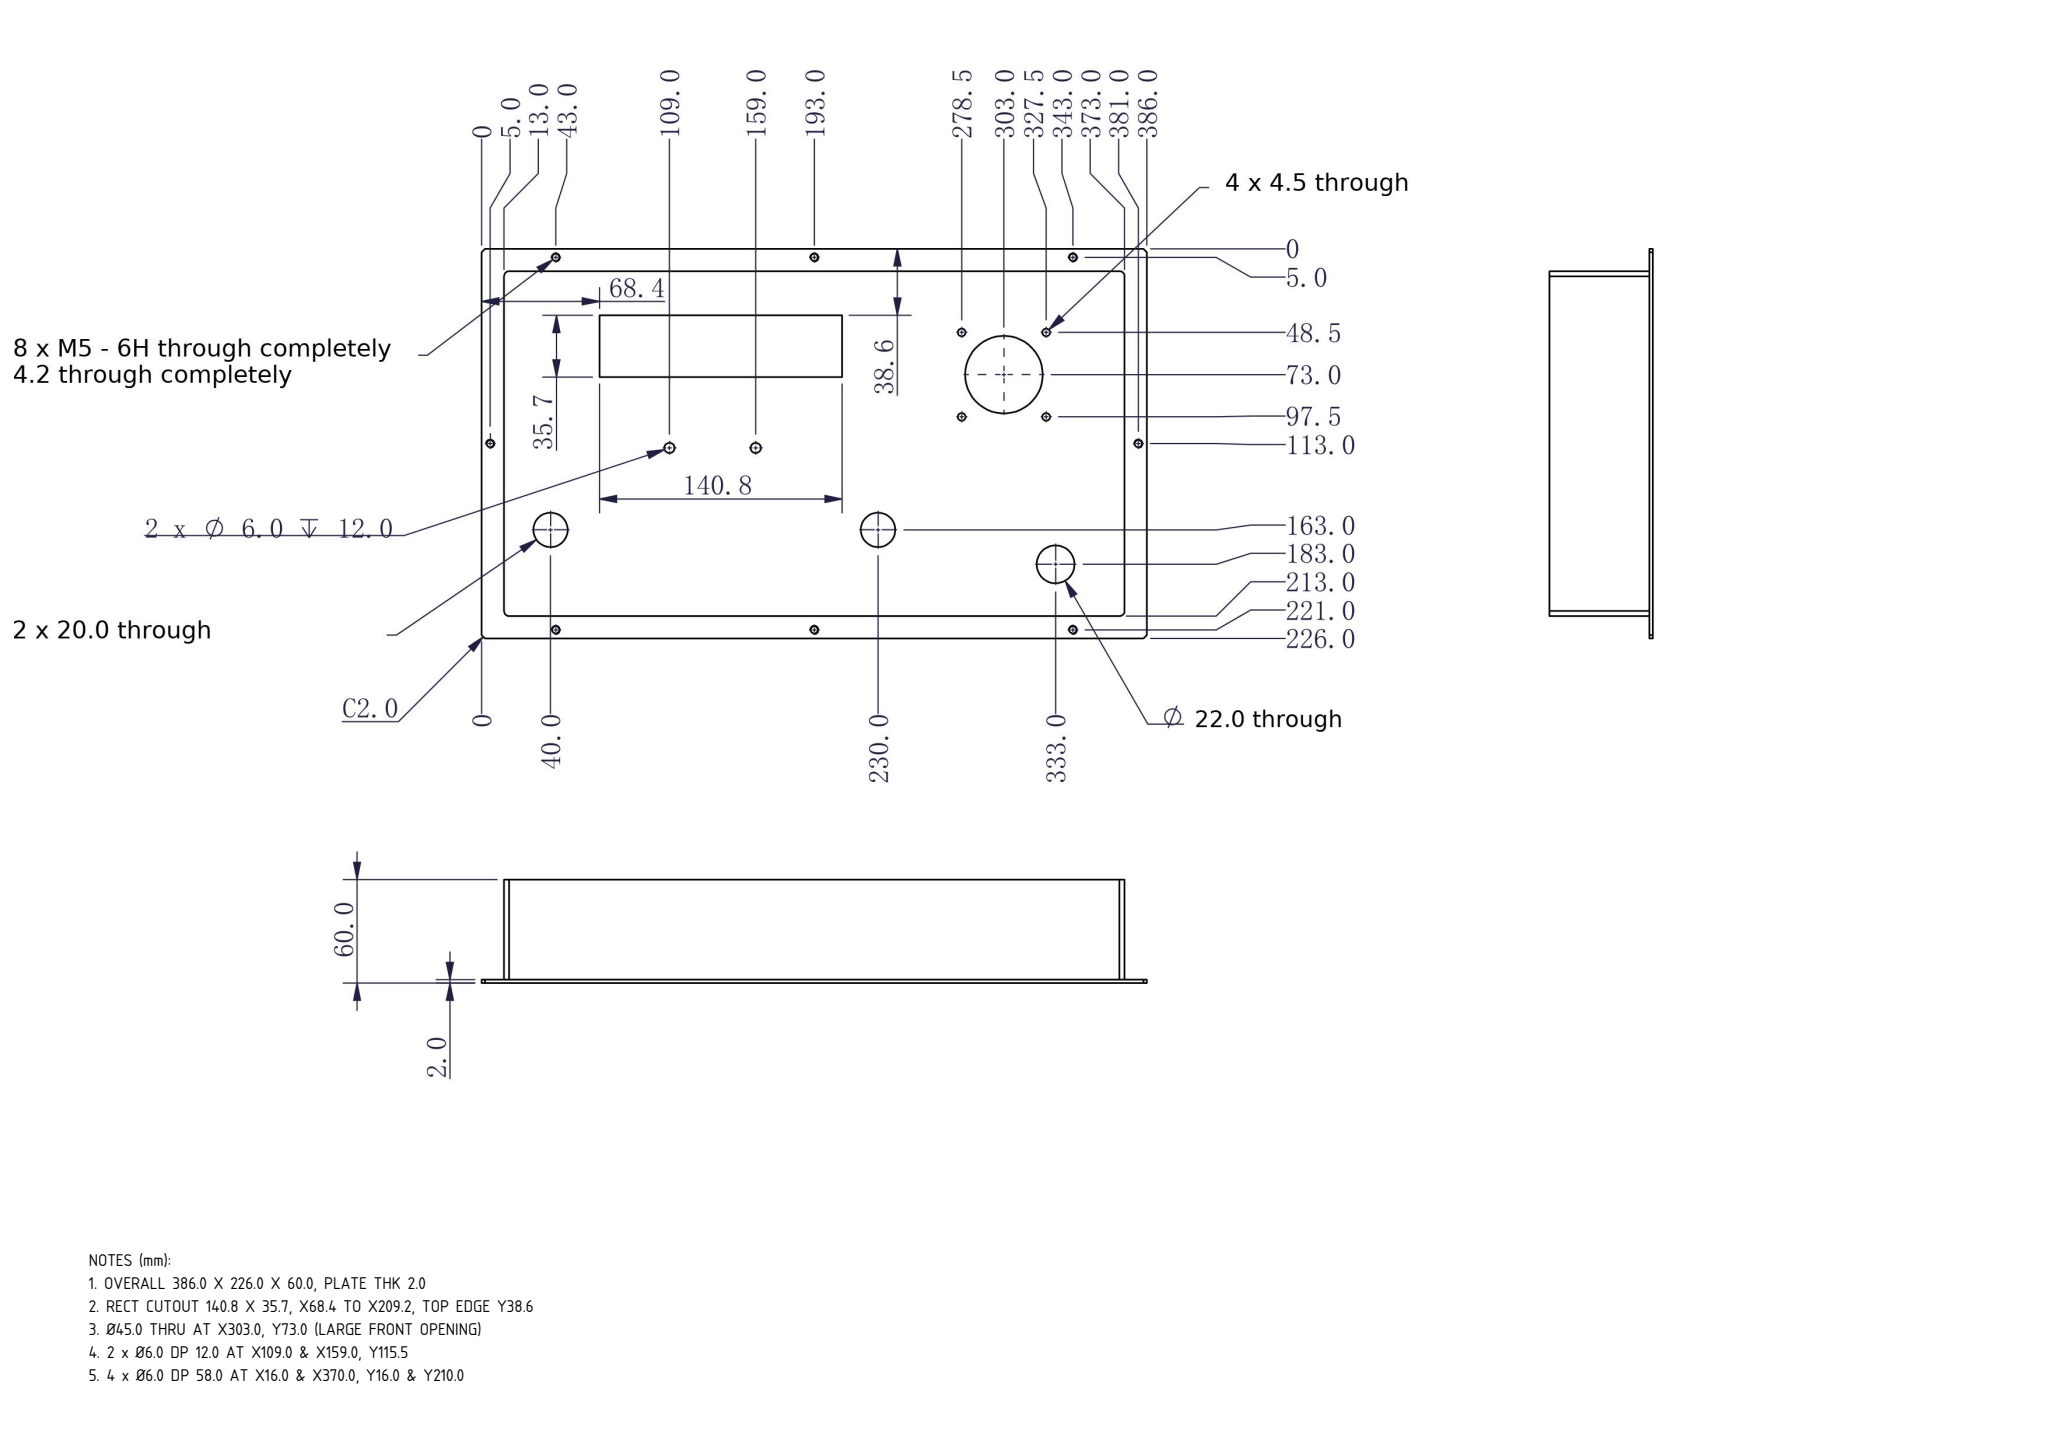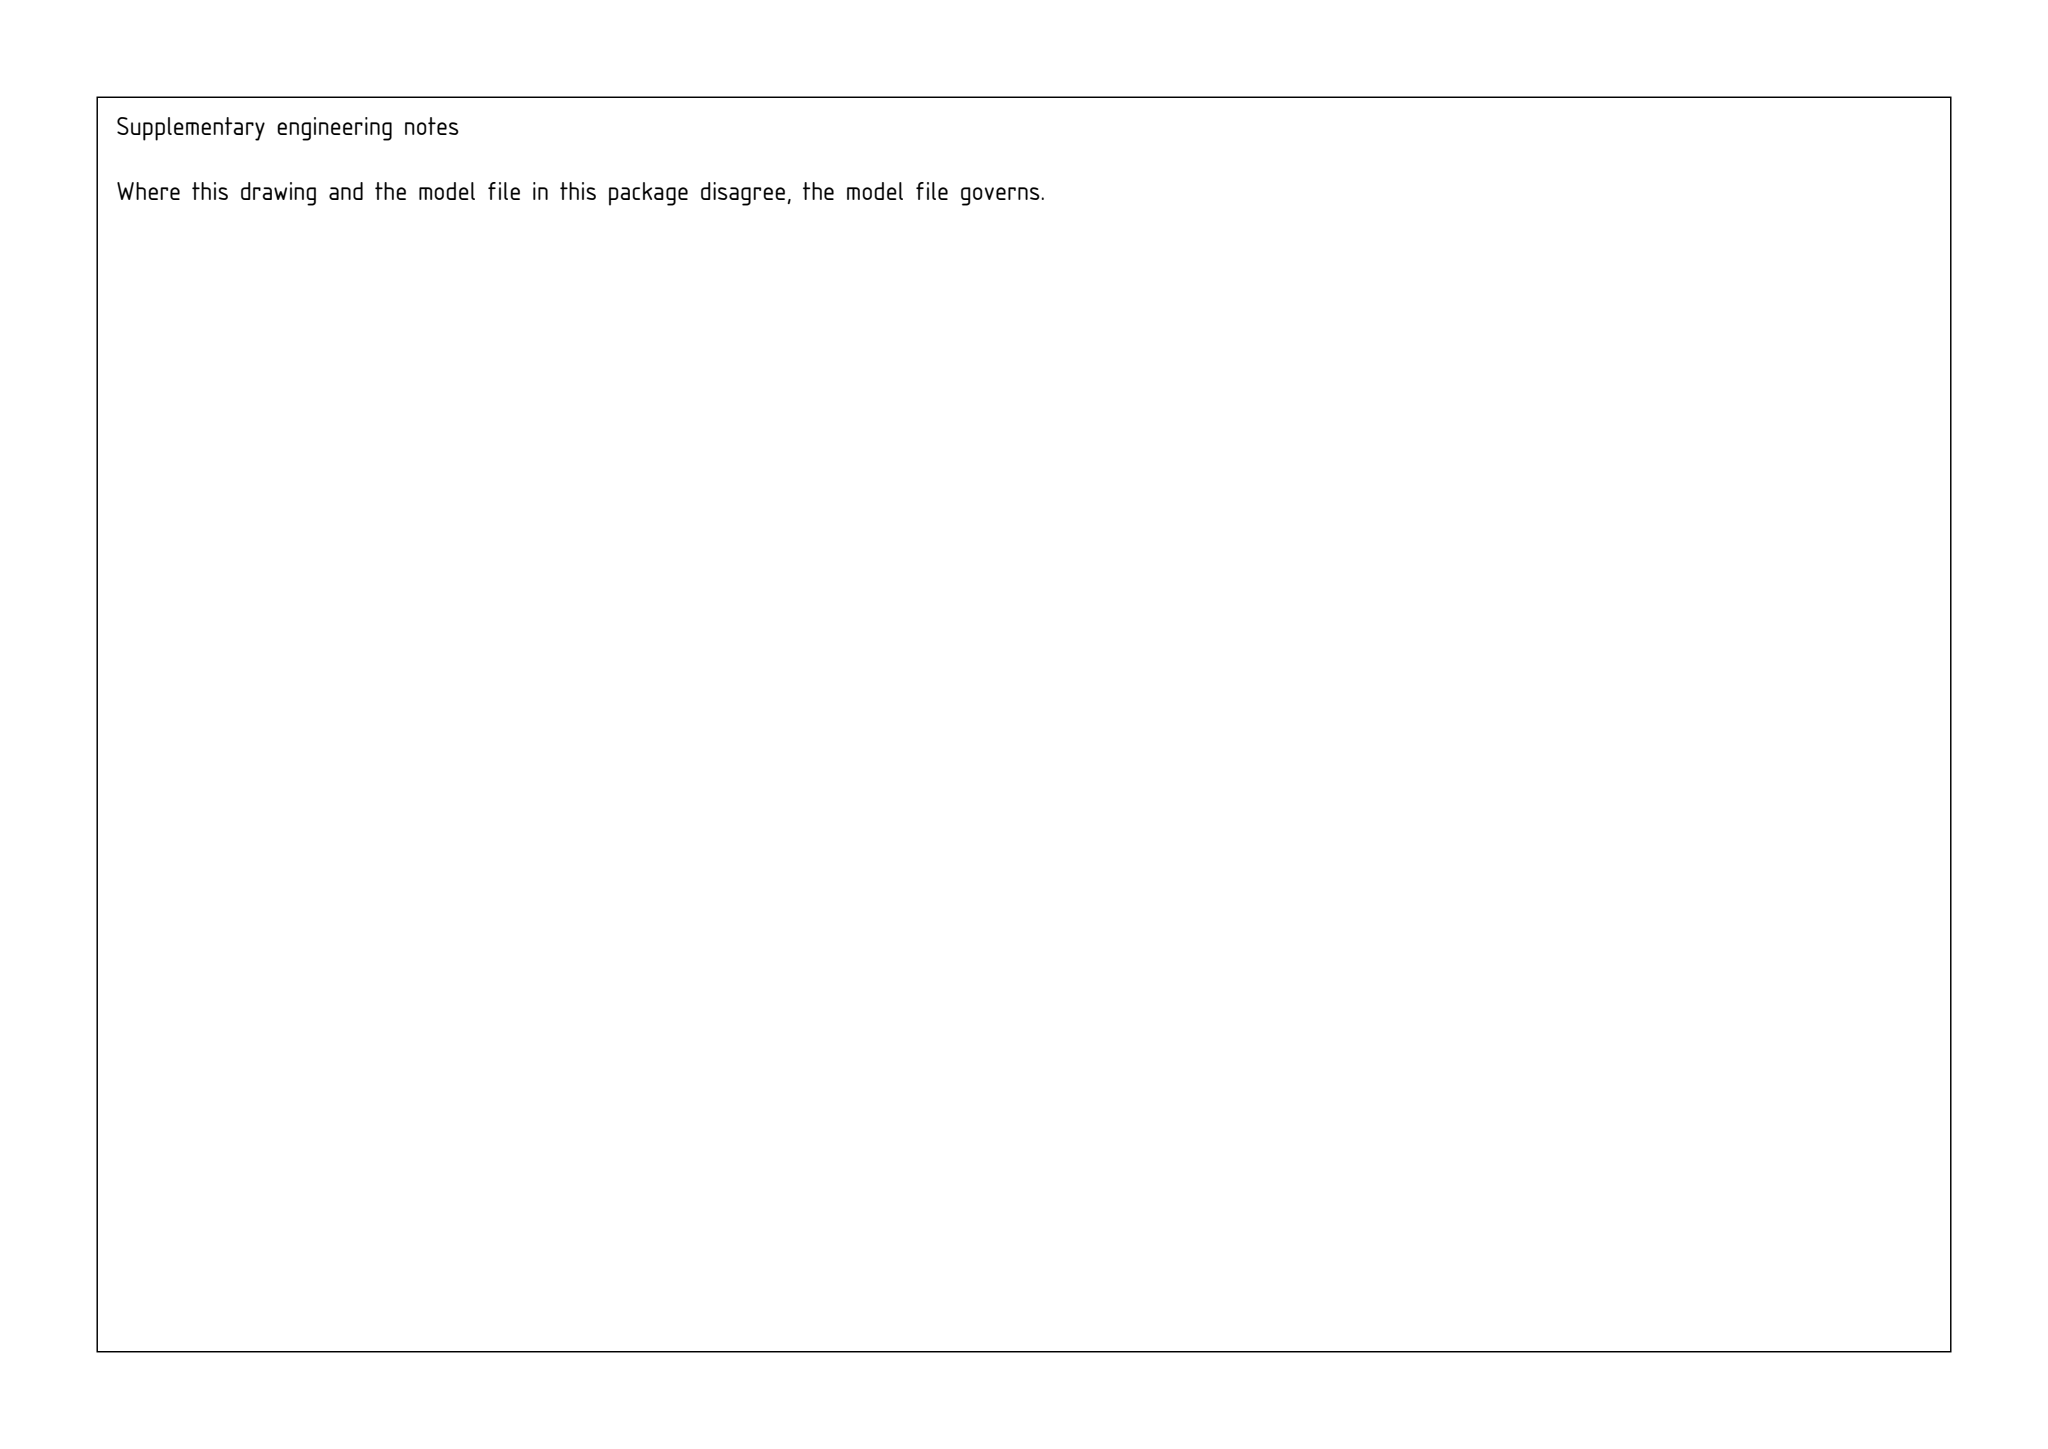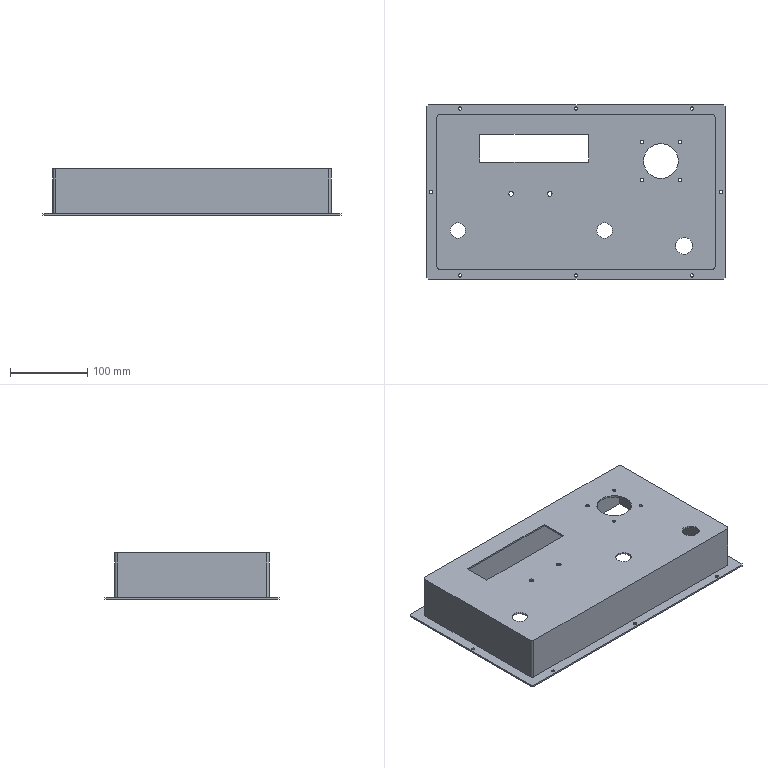Part | SolidWorks | mm | 1 solid | 64 faces | box 386 x 226 x 60 mm | volume 287277 mm3 | cylinder 40 | plane 24 | commonest cylinder face diameters 4.2 x16 6 x8 4.5 x8 20 x4 22 x2 45 x2
Drawing notes:
OVERALL 386.0 X 226.0 X 60.0, PLATE THK 2.0 | from the solid: bbox 386.0 x 226.0 x 60.0; z planes 0/2.0 and 58.0/60.0
RECT CUTOUT 140.8 X 35.7, X68.4 TO X209.2, TOP EDGE Y38.6 | from the solid: x planes 68.38 & 209.19 (140.81); y planes 151.64 & 187.37 (35.73); 226-187.37=38.63
Ø45.0 THRU AT X303.0, Y73.0 (LARGE FRONT OPENING) | from the solid: cylinder dia 45.0 axis z at [303.0,153.0] len 2.0; 226-153=73.0 from top datum
2 x Ø6.0 DP 12.0 AT X109.0 & X159.0, Y115.5 | from the solid: Ø6.0 z-cyls at (109.0,110.5) & (159.0,110.5); 226-110.5=115.5
4 x Ø6.0 DP 58.0 AT X16.0 & X370.0, Y16.0 & Y210.0 | from the solid: Ø6.0 len 58.0 z-cyls at (16,16),(16,210),(370,16),(370,210)
build123d program:
from build123d import *

# Parameters (mm, degrees)
SKETCH1_W                    = 360
SKETCH1_H                    = 200
BOSS_EXTRUDE1_DEPTH          = 60
SHELL1_T                     = -2
SKETCH2_W                    = 360
SKETCH2_H                    = 15
SKETCH2_W_2                  = 15
SKETCH2_H_2                  = 20
BOSS_EXTRUDE2_DEPTH          = 2
FILLET2_R                    = 3
M5_TAPPED_HOLE1_D            = 4.2
SKETCH6_R                    = 22.5
SKETCH6_R_2                  = 2.25
CUT_EXTRUDE1_DEPTH           = 232.045
SKETCH7_R                    = 10
CUT_EXTRUDE2_DEPTH           = 232.045
SKETCH8_R                    = 11
CUT_EXTRUDE3_DEPTH           = 232.045
SKETCH12_W                   = 13
SKETCH12_H                   = 103
BOSS_EXTRUDE3_DEPTH          = 2
CHAMFER1_SIZE                = 2
F_6_0_6_DIAMETER_HOLE1_D     = 6
F_6_0_6_DIAMETER_HOLE1_DEPTH = 12
F_6_0_6_DIAMETER_HOLE1_TIP   = 1.803
SKETCH17_W                   = 140.804
SKETCH17_H                   = 35.736
CUT_EXTRUDE6_DEPTH           = 10


with BuildPart() as part:
    # Sketch1 → Boss-Extrude1 (new body)
    with BuildSketch(Plane.XY):
        Rectangle(SKETCH1_W, SKETCH1_H)
    extrude(amount=BOSS_EXTRUDE1_DEPTH)

    # Shell1
    shell1_openings = [part.faces().sort_by_distance(p)[0] for p in [
        (0, 0, 0),
    ]]
    offset(amount=SHELL1_T, openings=shell1_openings, kind=Kind.INTERSECTION)

    # Sketch2 → Boss-Extrude2 (add)
    with BuildSketch(Plane(origin=(0, 0, 0), x_dir=(-1, 0, 0), z_dir=(0, 0, -1))):
        with Locations((0, 105.5)):
            Rectangle(SKETCH2_W, SKETCH2_H)
        with Locations((0, -105.5)):
            Rectangle(SKETCH2_W, SKETCH2_H)
        with Locations((-185.5, 0)):
            Rectangle(SKETCH2_W_2, SKETCH2_H_2)
        with Locations((185.5, 0)):
            Rectangle(SKETCH2_W_2, SKETCH2_H_2)
    extrude(amount=-BOSS_EXTRUDE2_DEPTH)

    # Fillet2
    fillet2_edges = [part.edges().sort_by_distance(p)[0] for p in [
        (180, -100, 31),
        (-180, -100, 31),
        (-180, 100, 31),
        (180, 100, 31),
    ]]
    fillet(fillet2_edges, radius=FILLET2_R)

    # M5 Tapped Hole1 (through all)
    with Locations(Plane(origin=(0, 0, 0), x_dir=(-1, 0, 0), z_dir=(0, 0, -1))):
        with Locations((-150, 108), (-188, 0), (150, 108), (188, 0), (150, -108), (-150, -108), (0, 108), (0, -108)):
            Hole(M5_TAPPED_HOLE1_D / 2)

    # Sketch6 → Cut-Extrude1 (cut, through all)
    with BuildSketch(Plane(origin=(0, 0, 58), x_dir=(-1, 0, 0), z_dir=(0, 0, -1))):
        with Locations((-110, 40)):
            Circle(SKETCH6_R)
        with Locations((-134.5, 15.5)):
            Circle(SKETCH6_R_2)
        with Locations(Location((-85.5, 15.5, 0), (0, 0, 180))):
            Circle(SKETCH6_R_2)
        with Locations((-85.5, 64.5)):
            Circle(SKETCH6_R_2)
        with Locations(Location((-134.5, 64.5, 0), (0, 0, 180))):
            Circle(SKETCH6_R_2)
    extrude(amount=-CUT_EXTRUDE1_DEPTH, mode=Mode.SUBTRACT)

    # Sketch7 → Cut-Extrude2 (cut, through all)
    with BuildSketch(Plane(origin=(0, 0, 58), x_dir=(-1, 0, 0), z_dir=(0, 0, -1))):
        with Locations((-37, -50)):
            Circle(SKETCH7_R)
        with Locations((153, -50)):
            Circle(SKETCH7_R)
    extrude(amount=-CUT_EXTRUDE2_DEPTH, mode=Mode.SUBTRACT)

    # Sketch8 → Cut-Extrude3 (cut, through all)
    with BuildSketch(Plane(origin=(0, 0, 58), x_dir=(-1, 0, 0), z_dir=(0, 0, -1))):
        with Locations((-140, -70)):
            Circle(SKETCH8_R)
    extrude(amount=-CUT_EXTRUDE3_DEPTH, mode=Mode.SUBTRACT)

    # Sketch12 → Boss-Extrude3 (add)
    with BuildSketch(Plane(origin=(0, 0, 0), x_dir=(-1, 0, 0), z_dir=(0, 0, -1))):
        with Locations((-186.5, 61.5)):
            Rectangle(SKETCH12_W, SKETCH12_H)
        with Locations((-186.5, -61.5)):
            Rectangle(SKETCH12_W, SKETCH12_H)
        with Locations((186.5, -61.5)):
            Rectangle(SKETCH12_W, SKETCH12_H)
        with Locations((186.5, 61.5)):
            Rectangle(SKETCH12_W, SKETCH12_H)
    extrude(amount=-BOSS_EXTRUDE3_DEPTH)

    # Chamfer1
    chamfer1_edges = [part.edges().sort_by_distance(p)[0] for p in [
        (193, 113, 1),
        (193, -113, 1),
        (-193, -113, 1),
        (-193, 113, 1),
    ]]
    chamfer(chamfer1_edges, length=CHAMFER1_SIZE)

    # 6.0 _6_ Diameter Hole1
    with Locations(Plane(origin=(0, 0, 58), x_dir=(-1, 0, 0), z_dir=(0, 0, -1))):
        with Locations((34, -2.5), (84, -2.5)):
            Hole(F_6_0_6_DIAMETER_HOLE1_D / 2, depth=F_6_0_6_DIAMETER_HOLE1_DEPTH)
            with Locations((0, 0, -(F_6_0_6_DIAMETER_HOLE1_DEPTH + F_6_0_6_DIAMETER_HOLE1_TIP / 2))):  # 118° drill point
                Cone(0, F_6_0_6_DIAMETER_HOLE1_D / 2, F_6_0_6_DIAMETER_HOLE1_TIP, mode=Mode.SUBTRACT)

    # Sketch17 → Cut-Extrude6 (cut)
    with BuildSketch(Plane(origin=(0, 0, 58), x_dir=(-1, 0, 0), z_dir=(0, 0, -1))):
        with Locations((54.214, 56.505)):
            Rectangle(SKETCH17_W, SKETCH17_H)
    extrude(amount=-CUT_EXTRUDE6_DEPTH, mode=Mode.SUBTRACT)


solid = part.part